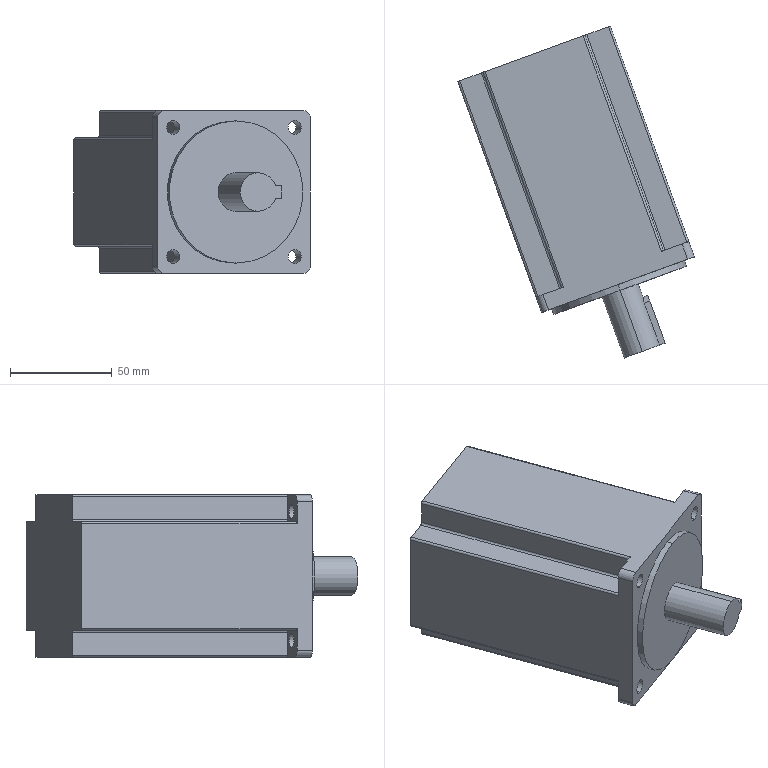Component | SolidWorks | AC1-08M30HC0A1-1 | 1 solid | 52 faces | volume 713638 mm3 | cylinder 29 | plane 23 | commonest cylinder face diameters 7 x12 2 x12 70 x2 19 x2 6 x1